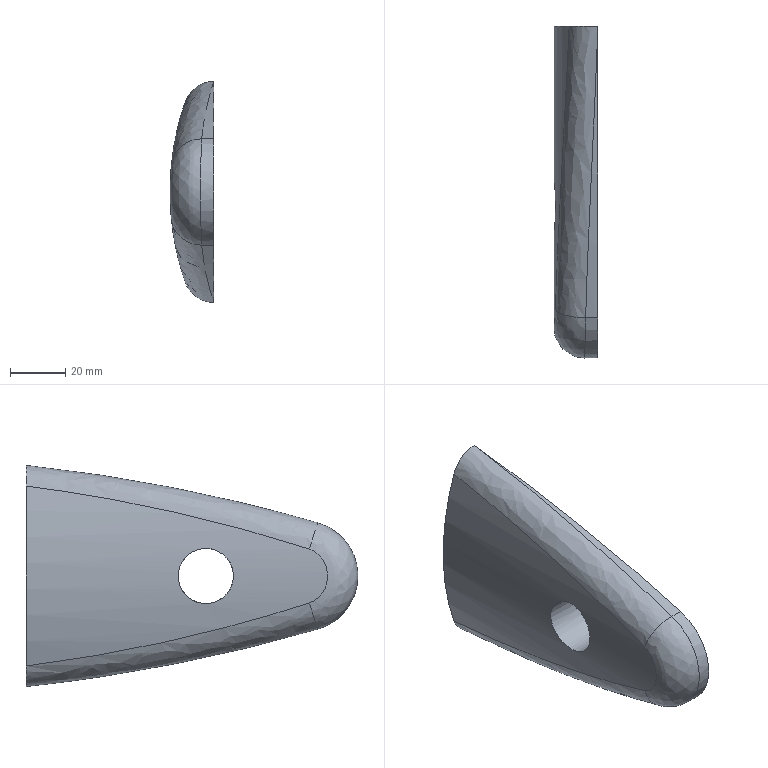Component | NX | FRONT_CASING | 1 solid | 25 faces | volume 25077 mm3 | cylinder 12 | spline 6 | plane 5 | other 2 | commonest cylinder face diameters 1247.218 x2 1252.218 x2 195 x1 40 x1 200 x1 35 x1 197.1 x1 28 x1